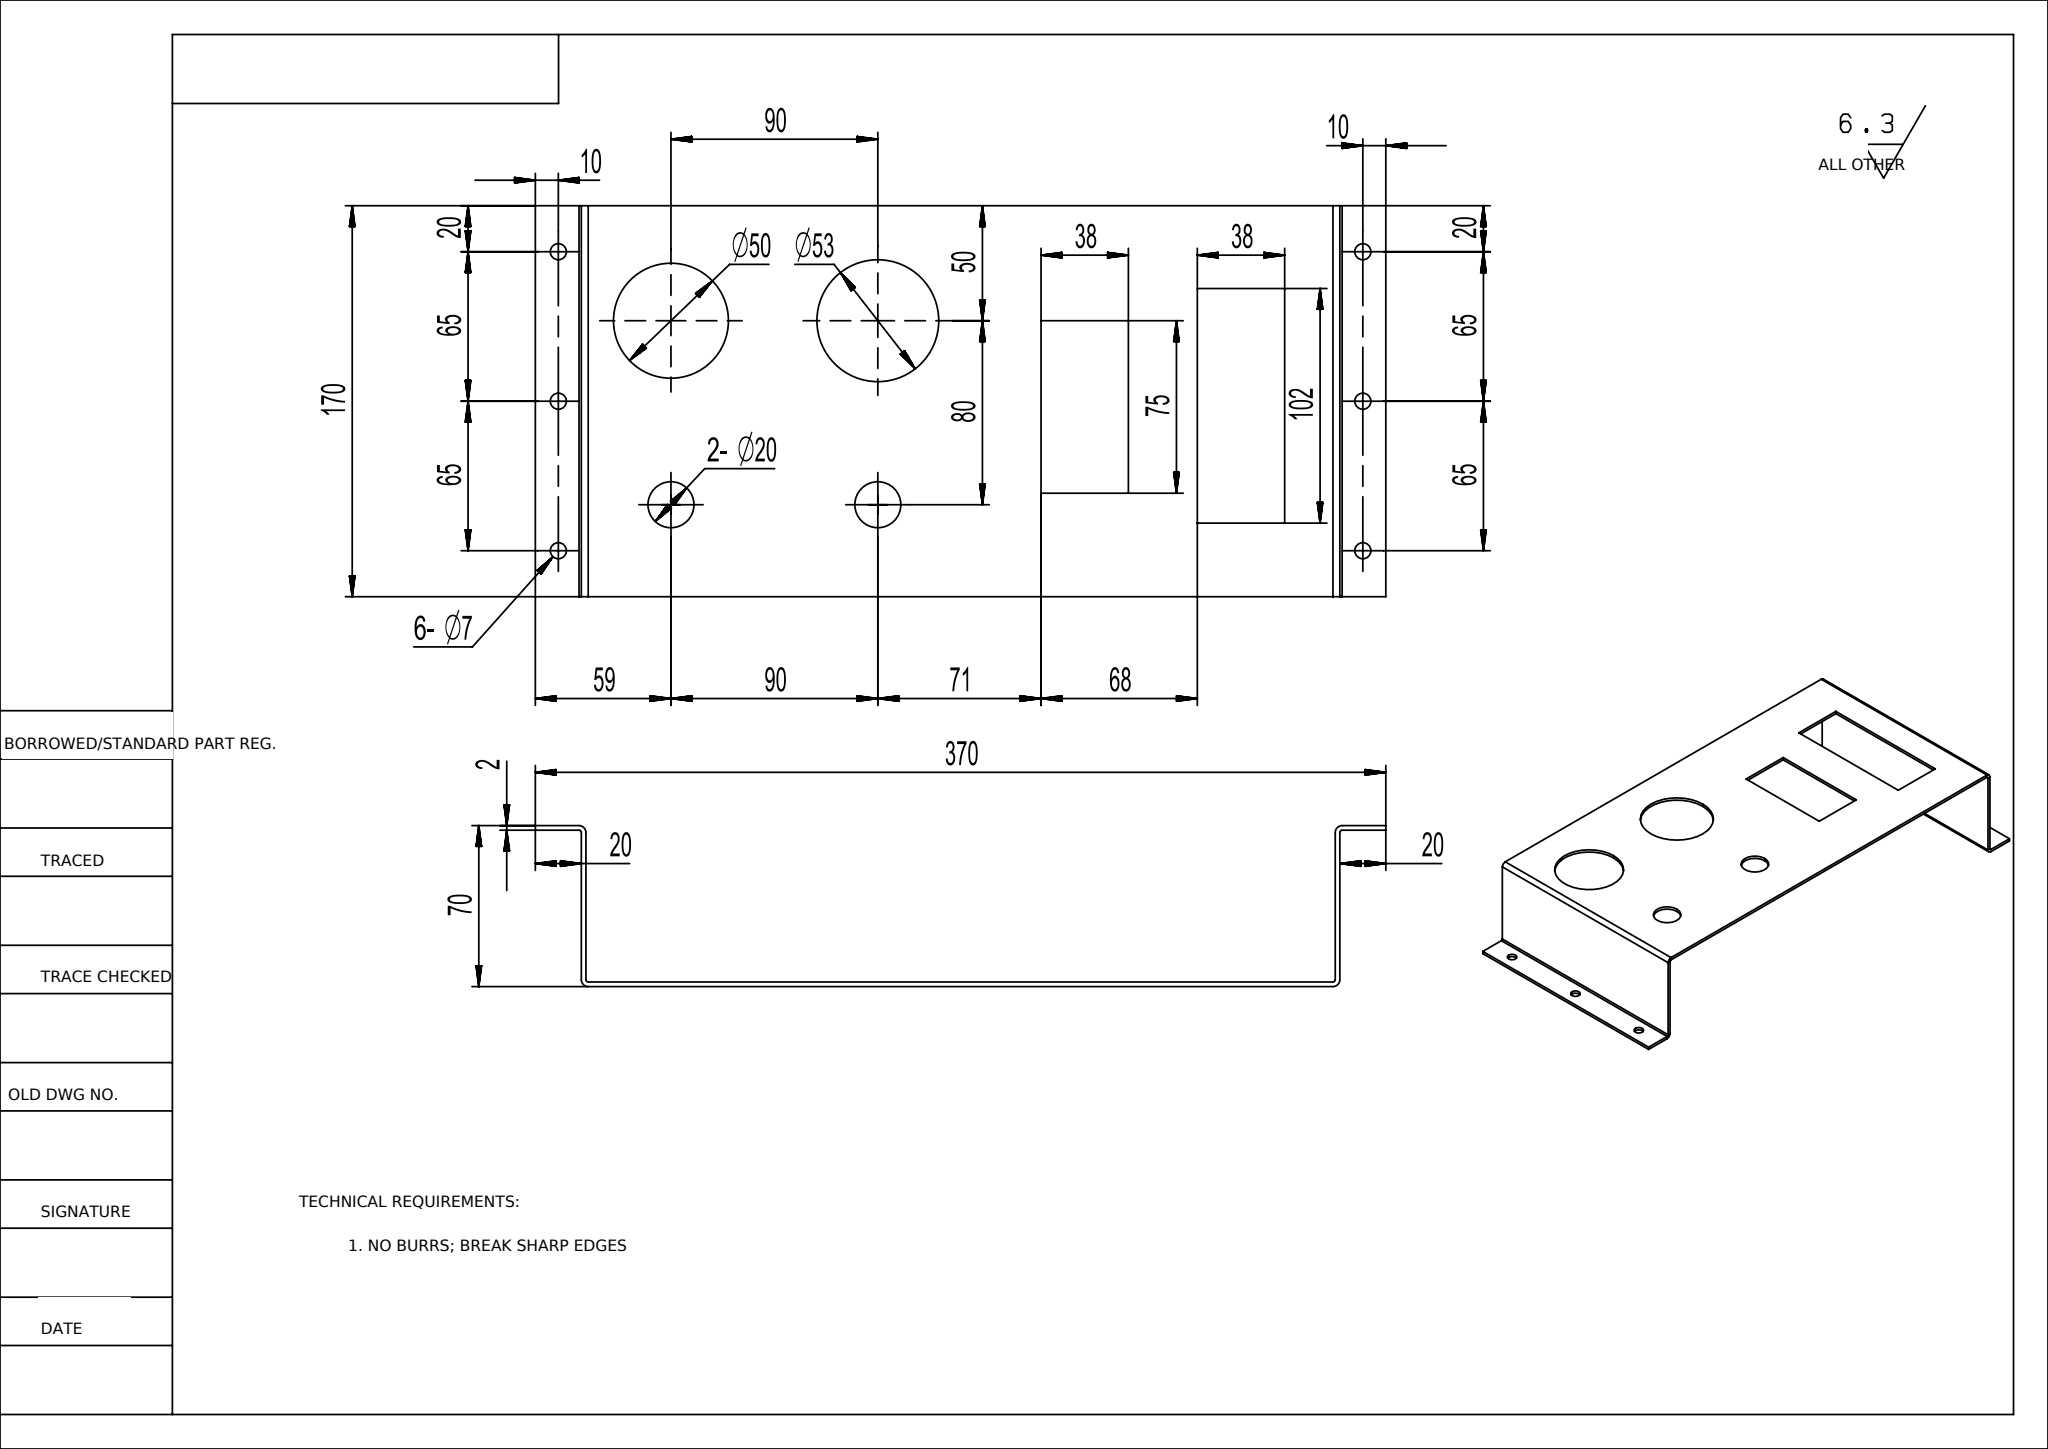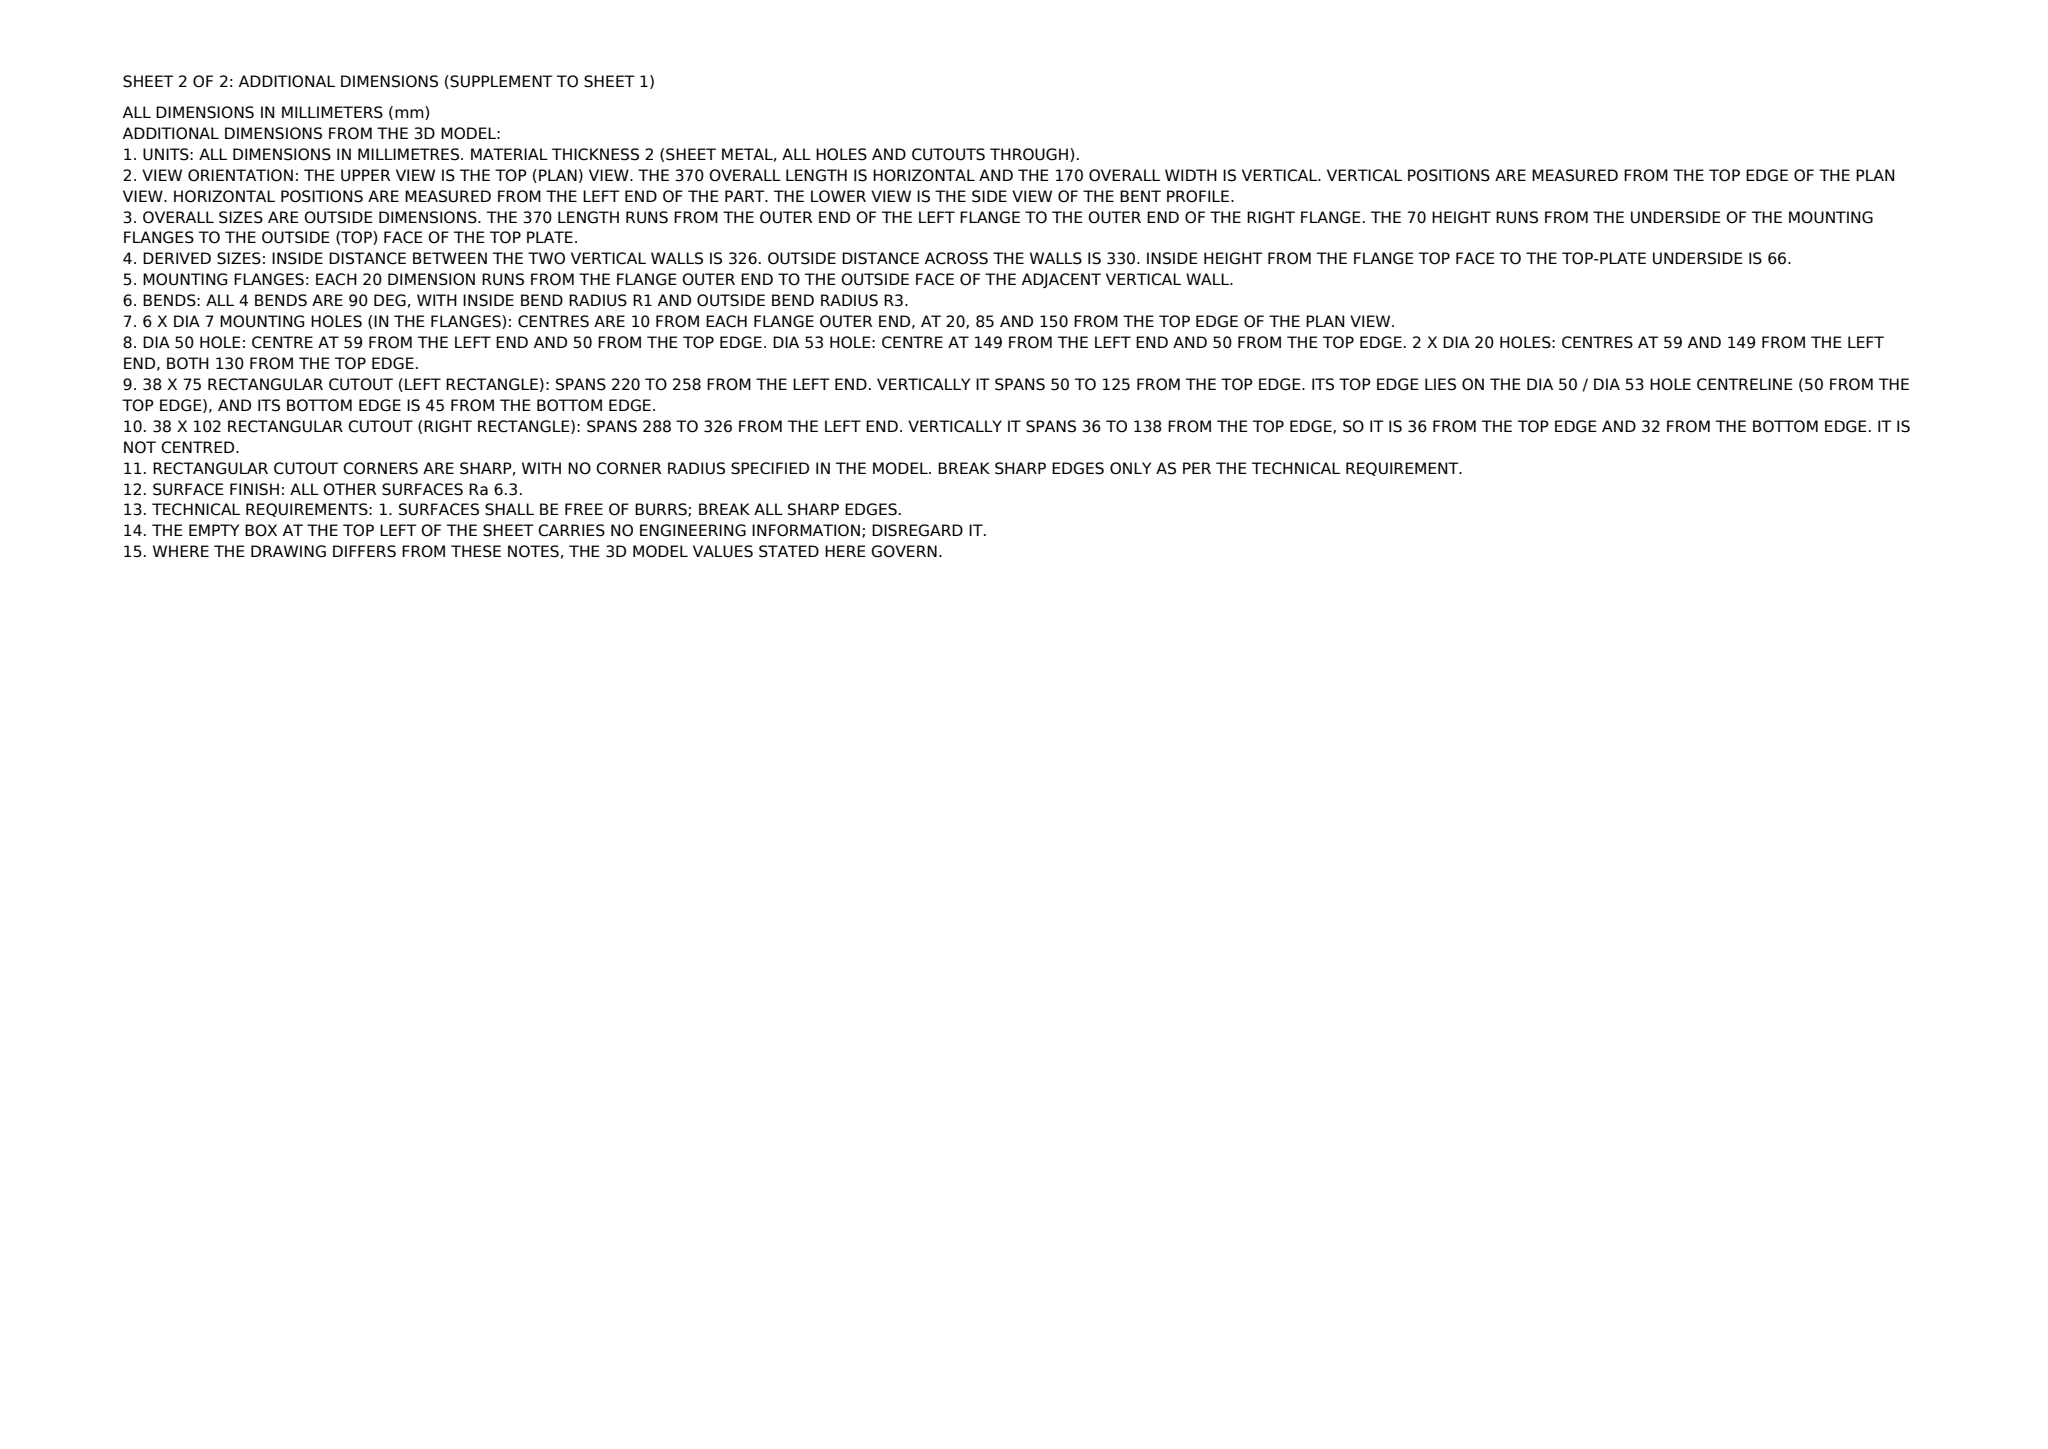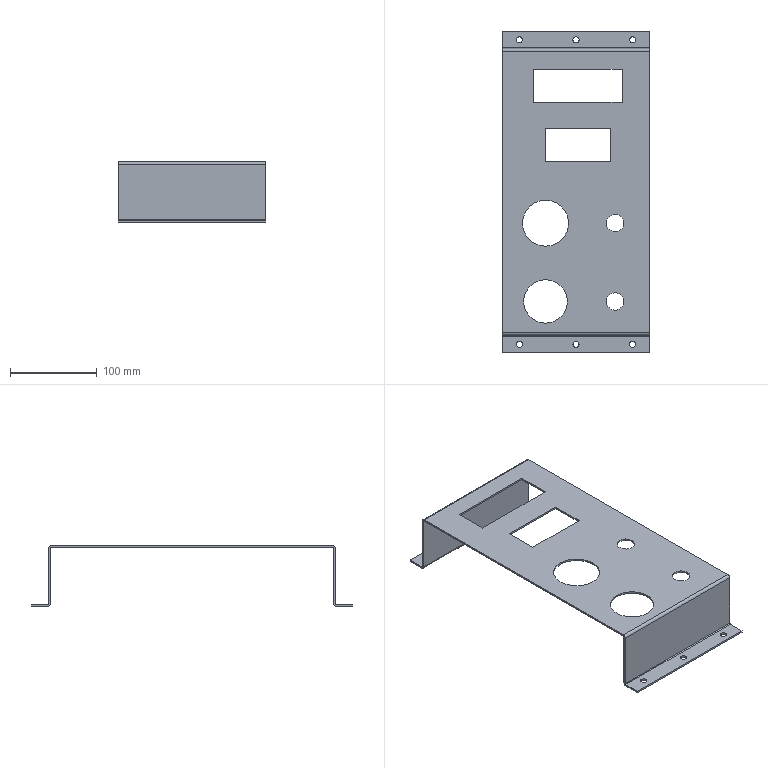Part | NX | mm | 1 solid | 40 faces | box 170 x 370 x 70 mm | volume 147363 mm3 | plane 22 | cylinder 18 | commonest cylinder face diameters 7 x6 2 x4 6 x4 20 x2 53 x1 50 x1